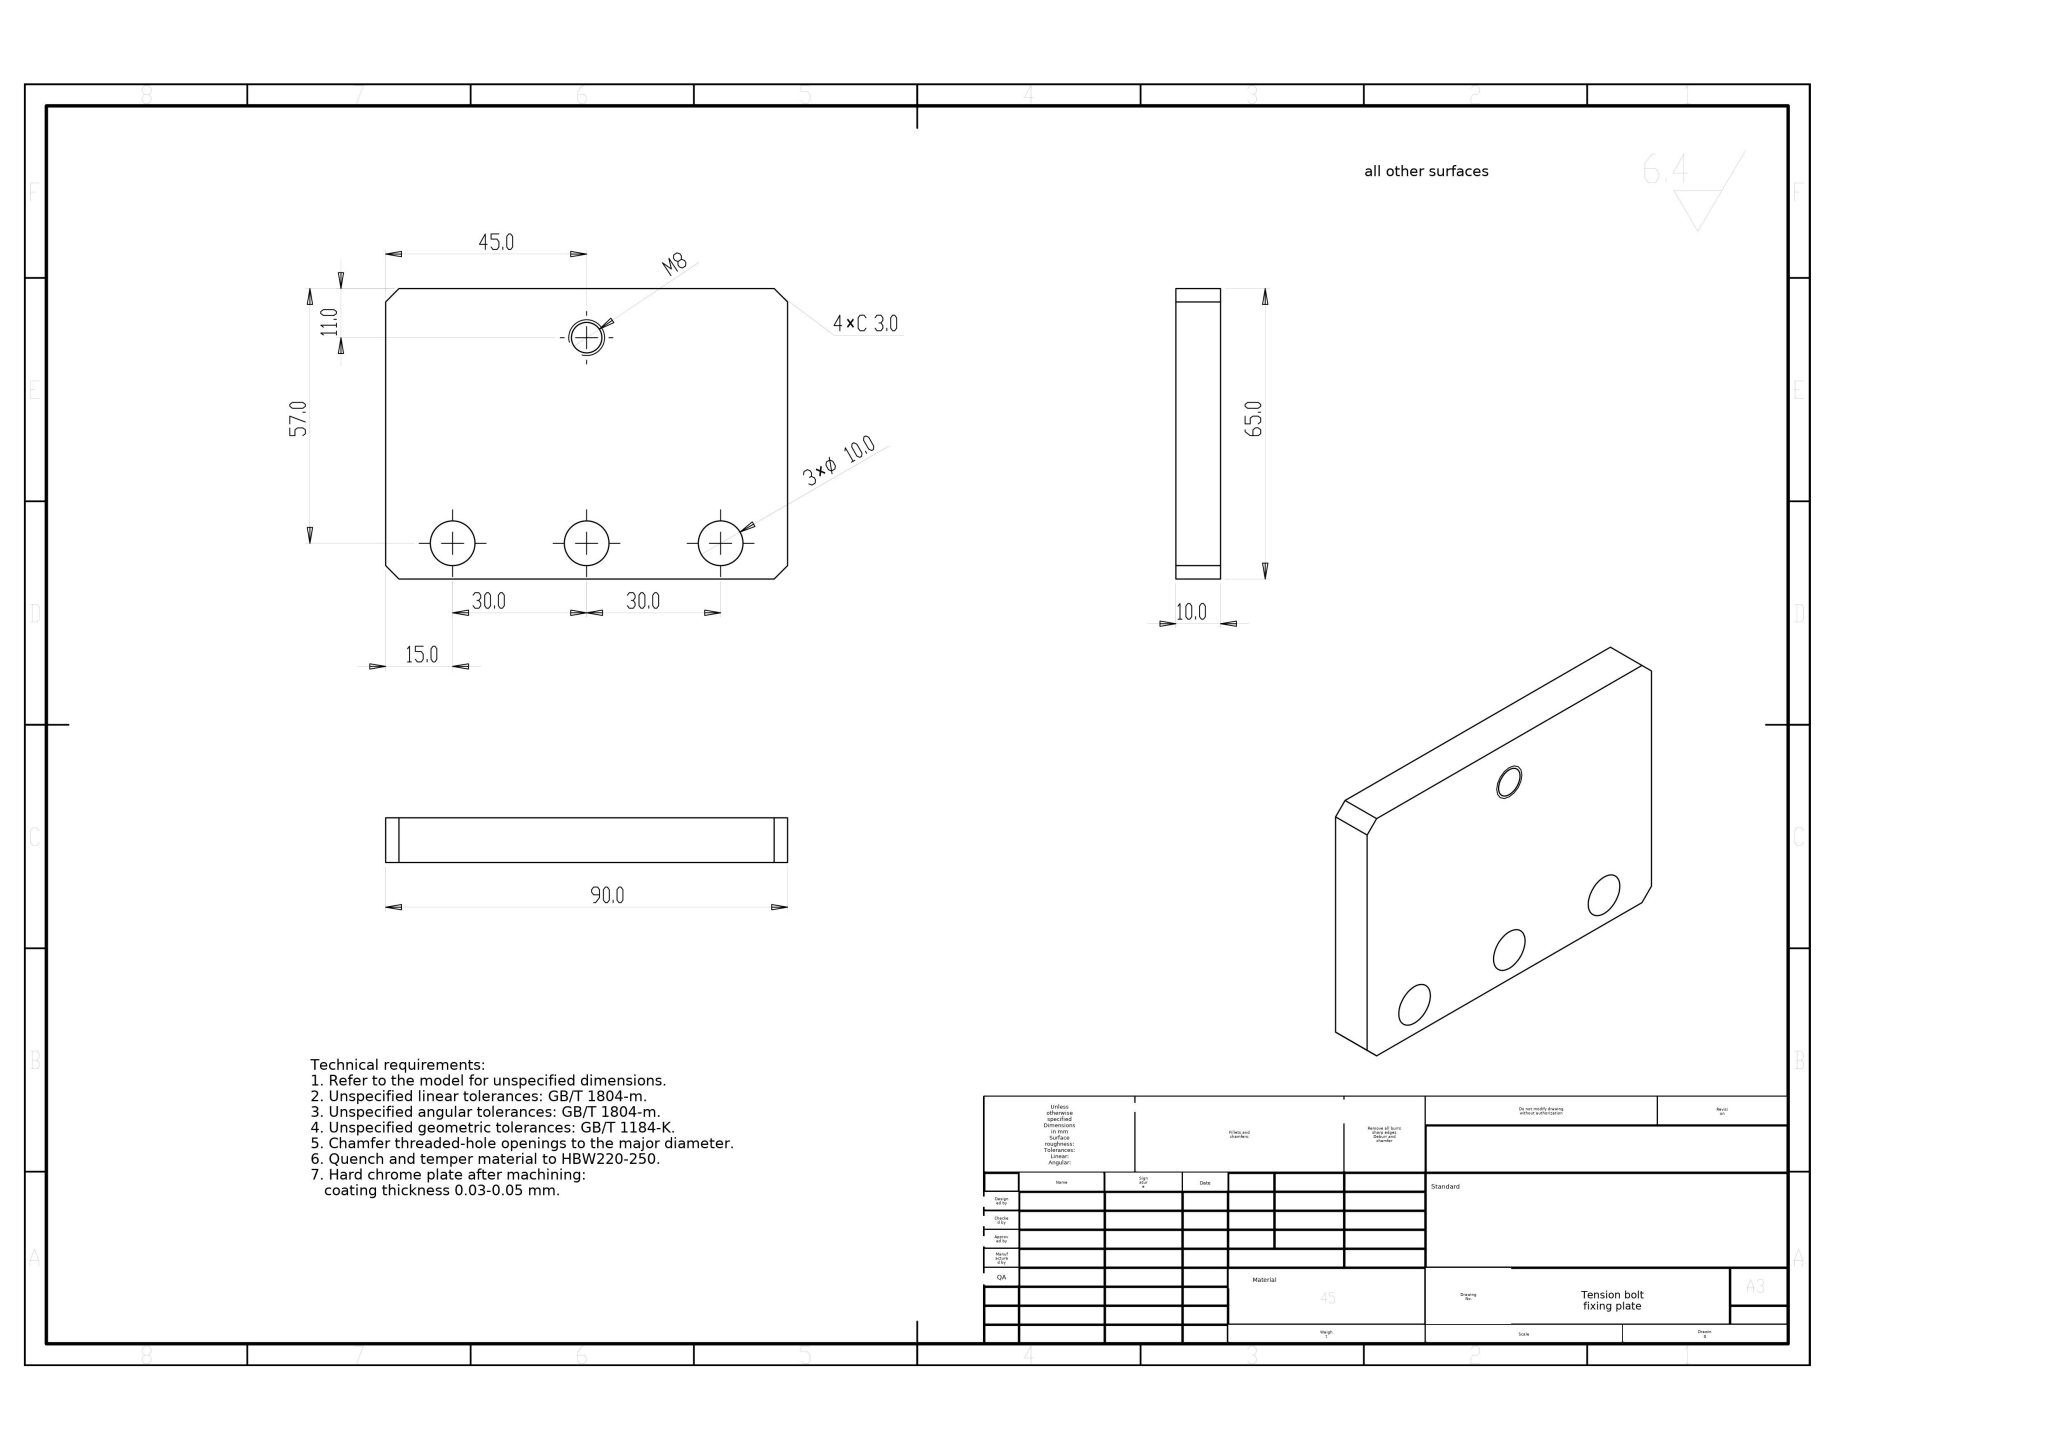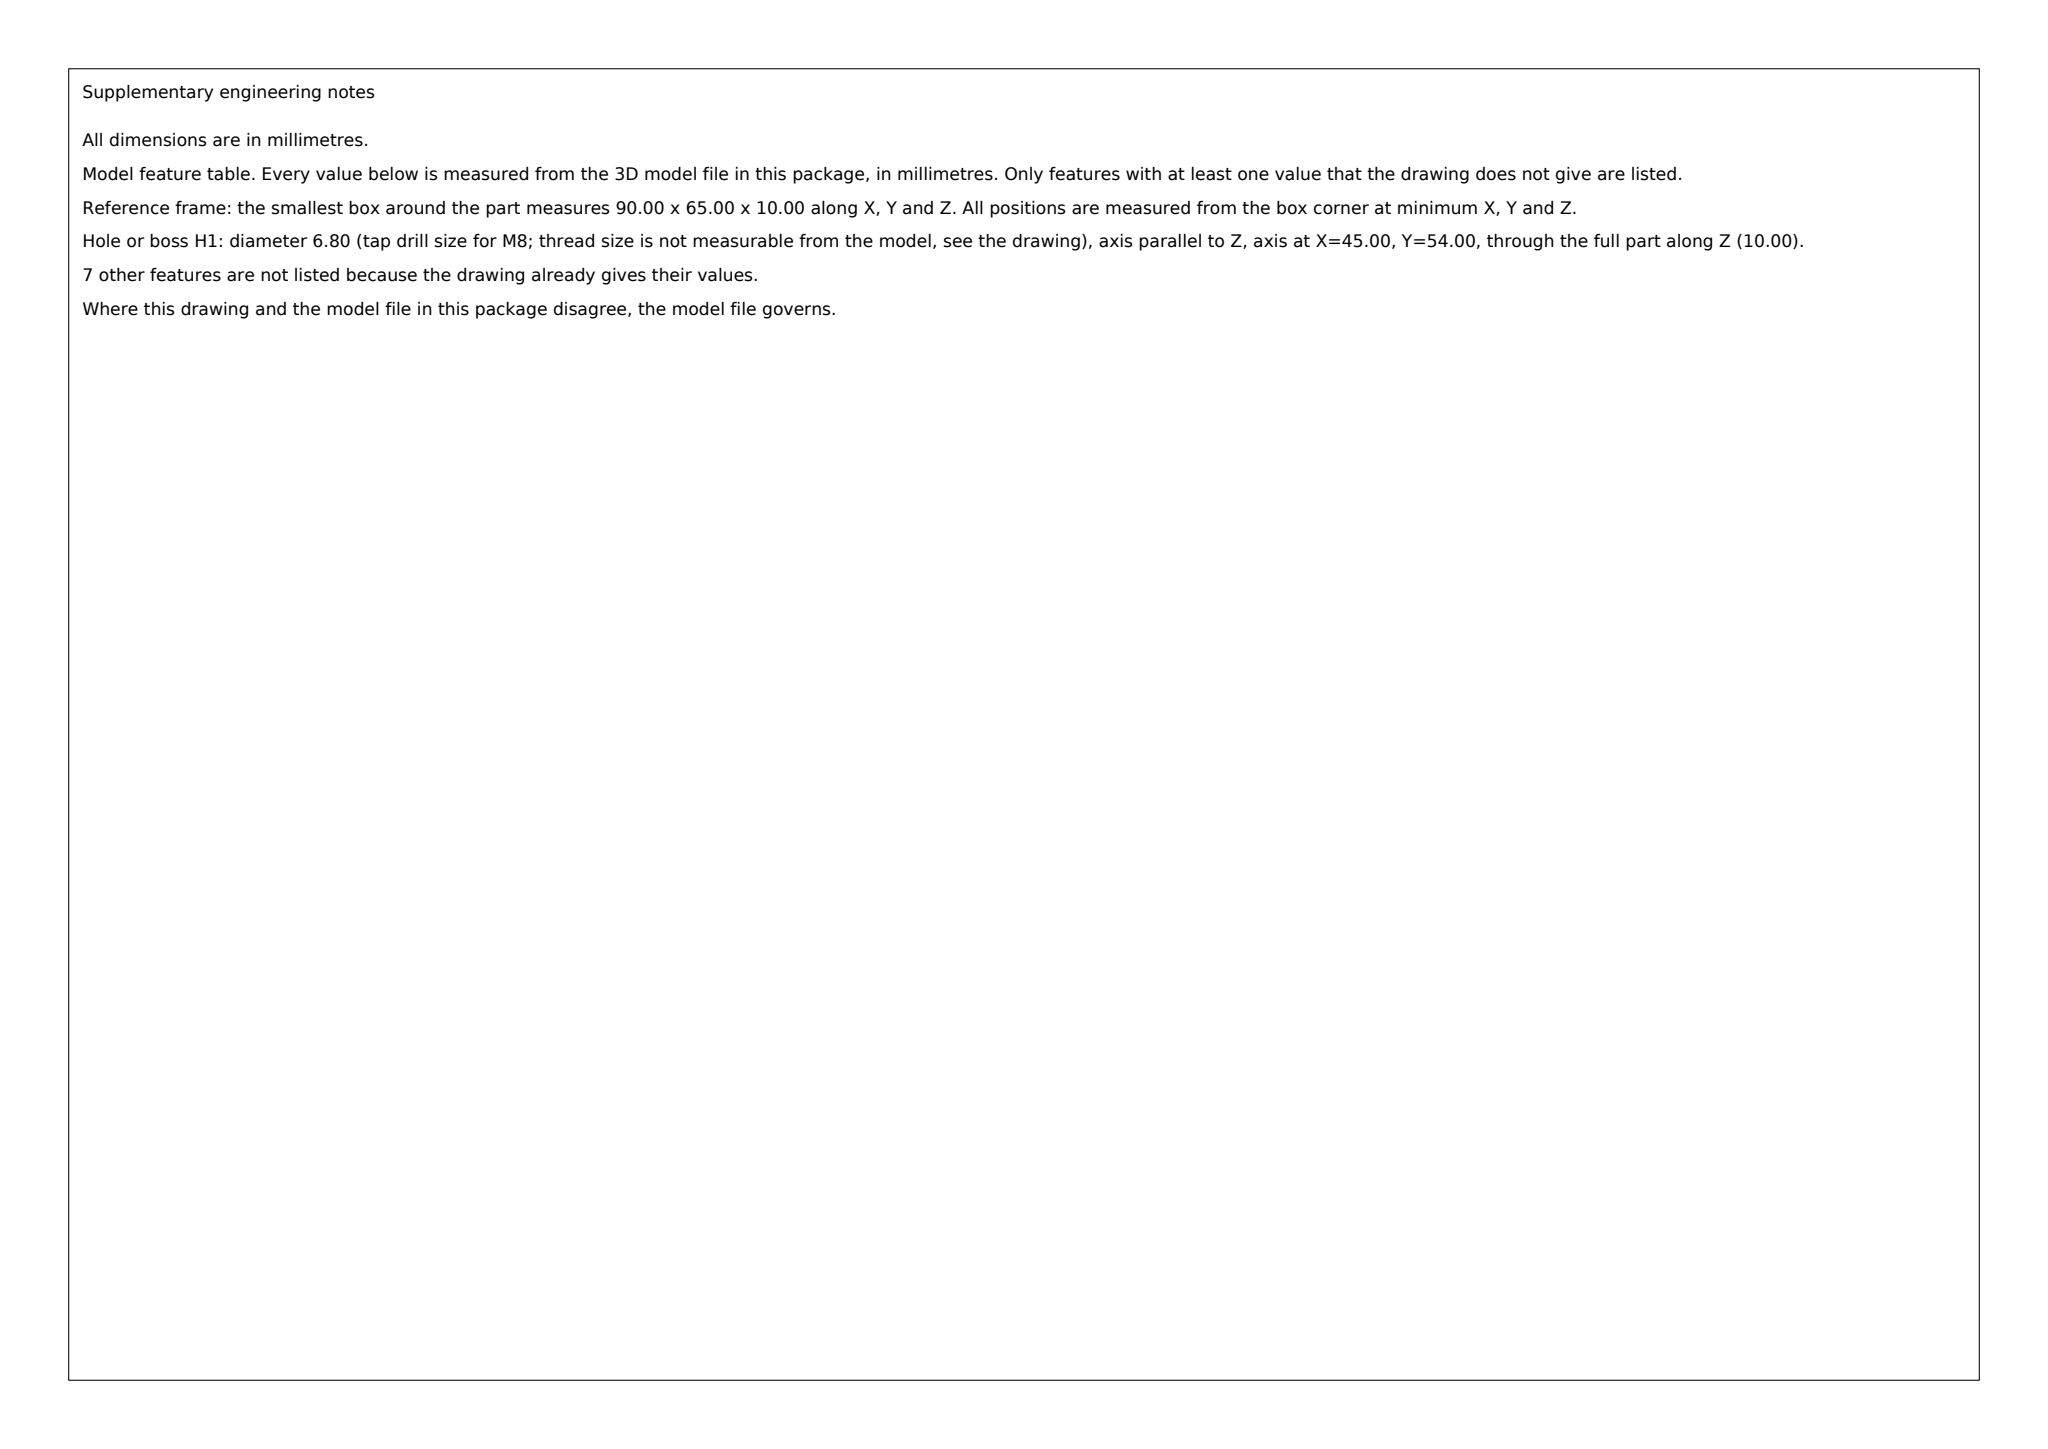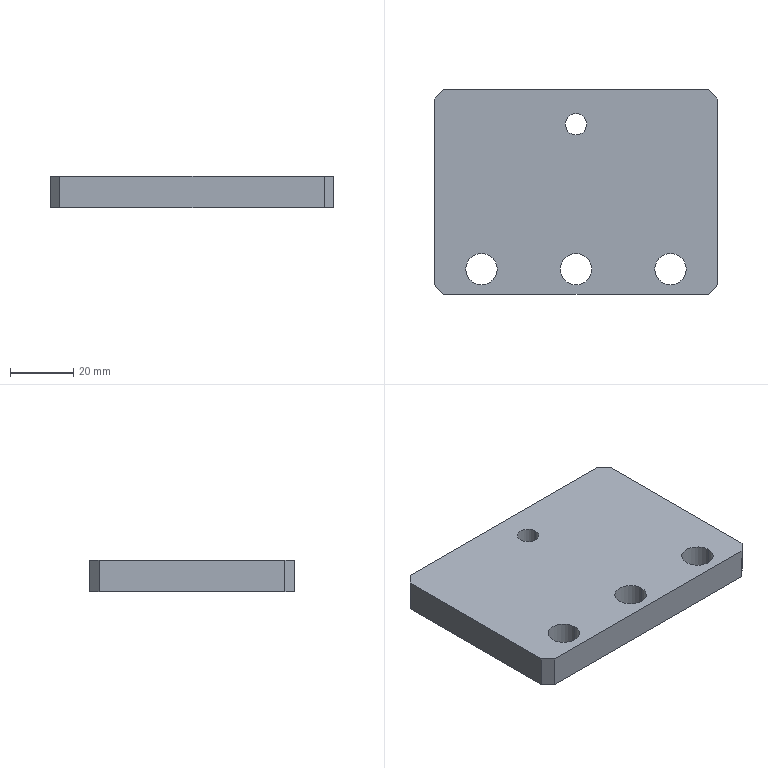Part | SolidWorks | mm | material 45 | 1 solid | 18 faces | box 90 x 65 x 10 mm | volume 55601 mm3 | plane 10 | cylinder 8 | commonest cylinder face diameters 10 x6 6.8 x2
build123d program:
from build123d import *

# Parameters (mm, degrees)
SKETCH1_W           = 90
SKETCH1_H           = 65
SKETCH1_R           = 5
BOSS_EXTRUDE1_DEPTH = 10
M8_TAPPED_HOLE1_D   = 6.8
CHAMFER1_SIZE       = 3


with BuildPart() as part:
    # Sketch1 → Boss-Extrude1 (new body)
    with BuildSketch(Plane.XY):
        with Locations((0, 24.5)):
            Rectangle(SKETCH1_W, SKETCH1_H)
        Circle(SKETCH1_R, mode=Mode.SUBTRACT)
        with Locations((30, 0)):
            Circle(SKETCH1_R, mode=Mode.SUBTRACT)
        with Locations(Location((-30, 0, 0), (0, 0, 180))):
            Circle(SKETCH1_R, mode=Mode.SUBTRACT)
    extrude(amount=BOSS_EXTRUDE1_DEPTH)

    # M8 Tapped Hole1 (through all)
    with Locations(Plane.XY.offset(10)):
        with Locations((0, 46)):
            Hole(M8_TAPPED_HOLE1_D / 2)

    # Chamfer1
    chamfer1_edges = [part.edges().sort_by_distance(p)[0] for p in [
        (45, -8, 5),
        (-45, -8, 5),
        (-45, 57, 5),
        (45, 57, 5),
    ]]
    chamfer(chamfer1_edges, length=CHAMFER1_SIZE)


solid = part.part
STEP:
#1=CARTESIAN_POINT('',(-3.4,46.,0.));
#2=VERTEX_POINT('',#1);
#3=CARTESIAN_POINT('',(3.4,46.,0.));
#4=VERTEX_POINT('',#3);
#5=CARTESIAN_POINT('',(0.,46.,0.));
#6=DIRECTION('',(0.,0.,1.));
#7=DIRECTION('',(1.,0.,0.));
#8=AXIS2_PLACEMENT_3D('',#5,#6,#7);
#9=CIRCLE('',#8,3.4);
#10=EDGE_CURVE('',#2,#4,#9,.T.);
#11=ORIENTED_EDGE('',*,*,#10,.F.);
#12=CARTESIAN_POINT('',(-3.4,46.,10.));
#13=VERTEX_POINT('',#12);
#14=CARTESIAN_POINT('',(-3.4,46.,10.));
#15=DIRECTION('',(0.,0.,1.));
#16=VECTOR('',#15,1000.);
#17=LINE('',#14,#16);
#18=EDGE_CURVE('',#2,#13,#17,.T.);
#19=ORIENTED_EDGE('',*,*,#18,.T.);
#20=CARTESIAN_POINT('',(3.4,46.,10.));
#21=VERTEX_POINT('',#20);
#22=CARTESIAN_POINT('',(0.,46.,10.));
#23=DIRECTION('',(0.,0.,1.));
#24=DIRECTION('',(1.,0.,0.));
#25=AXIS2_PLACEMENT_3D('',#22,#23,#24);
#26=CIRCLE('',#25,3.4);
#27=EDGE_CURVE('',#13,#21,#26,.T.);
#28=ORIENTED_EDGE('',*,*,#27,.T.);
#29=CARTESIAN_POINT('',(3.4,46.,10.));
#30=DIRECTION('',(0.,0.,1.));
#31=VECTOR('',#30,1000.);
#32=LINE('',#29,#31);
#33=EDGE_CURVE('',#4,#21,#32,.T.);
#34=ORIENTED_EDGE('',*,*,#33,.F.);
#35=EDGE_LOOP('',(#11,#19,#28,#34));
#36=FACE_OUTER_BOUND('',#35,.T.);
#37=CARTESIAN_POINT('',(0.,46.,10.));
#38=DIRECTION('',(0.,0.,1.));
#39=DIRECTION('',(1.,0.,0.));
#40=AXIS2_PLACEMENT_3D('',#37,#38,#39);
#41=CYLINDRICAL_SURFACE('',#40,3.4);
#42=ADVANCED_FACE('',(#36),#41,.F.);
#43=CARTESIAN_POINT('',(-35.,-0.,10.));
#44=VERTEX_POINT('',#43);
#45=CARTESIAN_POINT('',(-25.,-0.,10.));
#46=VERTEX_POINT('',#45);
#47=CARTESIAN_POINT('',(-30.,-0.,10.));
#48=DIRECTION('',(0.,0.,1.));
#49=DIRECTION('',(-1.,0.,0.));
#50=AXIS2_PLACEMENT_3D('',#47,#48,#49);
#51=CIRCLE('',#50,5.);
#52=EDGE_CURVE('',#44,#46,#51,.T.);
#53=ORIENTED_EDGE('',*,*,#52,.T.);
#54=CARTESIAN_POINT('',(-25.,-0.,0.));
#55=VERTEX_POINT('',#54);
#56=CARTESIAN_POINT('',(-25.,-0.,10.));
#57=DIRECTION('',(0.,0.,-1.));
#58=VECTOR('',#57,1000.);
#59=LINE('',#56,#58);
#60=EDGE_CURVE('',#46,#55,#59,.T.);
#61=ORIENTED_EDGE('',*,*,#60,.T.);
#62=CARTESIAN_POINT('',(-35.,-0.,0.));
#63=VERTEX_POINT('',#62);
#64=CARTESIAN_POINT('',(-30.,-0.,0.));
#65=DIRECTION('',(0.,0.,1.));
#66=DIRECTION('',(-1.,0.,0.));
#67=AXIS2_PLACEMENT_3D('',#64,#65,#66);
#68=CIRCLE('',#67,5.);
#69=EDGE_CURVE('',#63,#55,#68,.T.);
#70=ORIENTED_EDGE('',*,*,#69,.F.);
#71=CARTESIAN_POINT('',(-35.,-0.,10.));
#72=DIRECTION('',(0.,0.,-1.));
#73=VECTOR('',#72,1000.);
#74=LINE('',#71,#73);
#75=EDGE_CURVE('',#44,#63,#74,.T.);
#76=ORIENTED_EDGE('',*,*,#75,.F.);
#77=EDGE_LOOP('',(#53,#61,#70,#76));
#78=FACE_OUTER_BOUND('',#77,.T.);
#79=CARTESIAN_POINT('',(-30.,-0.,10.));
#80=DIRECTION('',(0.,0.,-1.));
#81=DIRECTION('',(-1.,0.,0.));
#82=AXIS2_PLACEMENT_3D('',#79,#80,#81);
#83=CYLINDRICAL_SURFACE('',#82,5.);
#84=ADVANCED_FACE('',(#78),#83,.F.);
#85=CARTESIAN_POINT('',(25.,0.,10.));
#86=VERTEX_POINT('',#85);
#87=CARTESIAN_POINT('',(35.,0.,10.));
#88=VERTEX_POINT('',#87);
#89=CARTESIAN_POINT('',(30.,0.,10.));
#90=DIRECTION('',(0.,0.,1.));
#91=DIRECTION('',(1.,0.,0.));
#92=AXIS2_PLACEMENT_3D('',#89,#90,#91);
#93=CIRCLE('',#92,5.);
#94=EDGE_CURVE('',#86,#88,#93,.T.);
#95=ORIENTED_EDGE('',*,*,#94,.T.);
#96=CARTESIAN_POINT('',(35.,0.,0.));
#97=VERTEX_POINT('',#96);
#98=CARTESIAN_POINT('',(35.,0.,10.));
#99=DIRECTION('',(0.,0.,-1.));
#100=VECTOR('',#99,1000.);
#101=LINE('',#98,#100);
#102=EDGE_CURVE('',#88,#97,#101,.T.);
#103=ORIENTED_EDGE('',*,*,#102,.T.);
#104=CARTESIAN_POINT('',(25.,0.,0.));
#105=VERTEX_POINT('',#104);
#106=CARTESIAN_POINT('',(30.,0.,0.));
#107=DIRECTION('',(0.,0.,1.));
#108=DIRECTION('',(1.,0.,0.));
#109=AXIS2_PLACEMENT_3D('',#106,#107,#108);
#110=CIRCLE('',#109,5.);
#111=EDGE_CURVE('',#105,#97,#110,.T.);
#112=ORIENTED_EDGE('',*,*,#111,.F.);
#113=CARTESIAN_POINT('',(25.,0.,10.));
#114=DIRECTION('',(0.,0.,-1.));
#115=VECTOR('',#114,1000.);
#116=LINE('',#113,#115);
#117=EDGE_CURVE('',#86,#105,#116,.T.);
#118=ORIENTED_EDGE('',*,*,#117,.F.);
#119=EDGE_LOOP('',(#95,#103,#112,#118));
#120=FACE_OUTER_BOUND('',#119,.T.);
#121=CARTESIAN_POINT('',(30.,0.,10.));
#122=DIRECTION('',(0.,0.,-1.));
#123=DIRECTION('',(-1.,0.,0.));
#124=AXIS2_PLACEMENT_3D('',#121,#122,#123);
#125=CYLINDRICAL_SURFACE('',#124,5.);
#126=ADVANCED_FACE('',(#120),#125,.F.);
#127=CARTESIAN_POINT('',(-5.,0.,10.));
#128=VERTEX_POINT('',#127);
#129=CARTESIAN_POINT('',(5.,0.,10.));
#130=VERTEX_POINT('',#129);
#131=CARTESIAN_POINT('',(0.,0.,10.));
#132=DIRECTION('',(0.,0.,1.));
#133=DIRECTION('',(1.,0.,0.));
#134=AXIS2_PLACEMENT_3D('',#131,#132,#133);
#135=CIRCLE('',#134,5.);
#136=EDGE_CURVE('',#128,#130,#135,.T.);
#137=ORIENTED_EDGE('',*,*,#136,.T.);
#138=CARTESIAN_POINT('',(5.,0.,0.));
#139=VERTEX_POINT('',#138);
#140=CARTESIAN_POINT('',(5.,0.,10.));
#141=DIRECTION('',(0.,0.,-1.));
#142=VECTOR('',#141,1000.);
#143=LINE('',#140,#142);
#144=EDGE_CURVE('',#130,#139,#143,.T.);
#145=ORIENTED_EDGE('',*,*,#144,.T.);
#146=CARTESIAN_POINT('',(-5.,0.,0.));
#147=VERTEX_POINT('',#146);
#148=CARTESIAN_POINT('',(0.,0.,0.));
#149=DIRECTION('',(0.,0.,1.));
#150=DIRECTION('',(1.,0.,0.));
#151=AXIS2_PLACEMENT_3D('',#148,#149,#150);
#152=CIRCLE('',#151,5.);
#153=EDGE_CURVE('',#147,#139,#152,.T.);
#154=ORIENTED_EDGE('',*,*,#153,.F.);
#155=CARTESIAN_POINT('',(-5.,0.,10.));
#156=DIRECTION('',(0.,0.,-1.));
#157=VECTOR('',#156,1000.);
#158=LINE('',#155,#157);
#159=EDGE_CURVE('',#128,#147,#158,.T.);
#160=ORIENTED_EDGE('',*,*,#159,.F.);
#161=EDGE_LOOP('',(#137,#145,#154,#160));
#162=FACE_OUTER_BOUND('',#161,.T.);
#163=CARTESIAN_POINT('',(0.,0.,10.));
#164=DIRECTION('',(0.,0.,-1.));
#165=DIRECTION('',(-1.,0.,0.));
#166=AXIS2_PLACEMENT_3D('',#163,#164,#165);
#167=CYLINDRICAL_SURFACE('',#166,5.);
#168=ADVANCED_FACE('',(#162),#167,.F.);
#169=CARTESIAN_POINT('',(0.,46.,10.));
#170=DIRECTION('',(0.,0.,1.));
#171=DIRECTION('',(1.,0.,0.));
#172=AXIS2_PLACEMENT_3D('',#169,#170,#171);
#173=CIRCLE('',#172,3.4);
#174=EDGE_CURVE('',#21,#13,#173,.T.);
#175=ORIENTED_EDGE('',*,*,#174,.F.);
#176=ORIENTED_EDGE('',*,*,#27,.F.);
#177=EDGE_LOOP('',(#175,#176));
#178=FACE_BOUND('',#177,.T.);
#179=ORIENTED_EDGE('',*,*,#94,.F.);
#180=CARTESIAN_POINT('',(30.,0.,10.));
#181=DIRECTION('',(0.,0.,1.));
#182=DIRECTION('',(1.,0.,0.));
#183=AXIS2_PLACEMENT_3D('',#180,#181,#182);
#184=CIRCLE('',#183,5.);
#185=EDGE_CURVE('',#88,#86,#184,.T.);
#186=ORIENTED_EDGE('',*,*,#185,.F.);
#187=EDGE_LOOP('',(#179,#186));
#188=FACE_BOUND('',#187,.T.);
#189=CARTESIAN_POINT('',(42.,57.,10.));
#190=VERTEX_POINT('',#189);
#191=CARTESIAN_POINT('',(-42.,57.,10.));
#192=VERTEX_POINT('',#191);
#193=CARTESIAN_POINT('',(-45.,57.,10.));
#194=DIRECTION('',(-1.,0.,0.));
#195=VECTOR('',#194,1000.);
#196=LINE('',#193,#195);
#197=EDGE_CURVE('',#190,#192,#196,.T.);
#198=ORIENTED_EDGE('',*,*,#197,.T.);
#199=CARTESIAN_POINT('',(-45.,54.,10.));
#200=VERTEX_POINT('',#199);
#201=CARTESIAN_POINT('',(-49.5,49.5,10.));
#202=DIRECTION('',(-0.7071,-0.7071,0.));
#203=VECTOR('',#202,1000.);
#204=LINE('',#201,#203);
#205=EDGE_CURVE('',#192,#200,#204,.T.);
#206=ORIENTED_EDGE('',*,*,#205,.T.);
#207=CARTESIAN_POINT('',(-45.,-5.,10.));
#208=VERTEX_POINT('',#207);
#209=CARTESIAN_POINT('',(-45.,57.,10.));
#210=DIRECTION('',(0.,-1.,0.));
#211=VECTOR('',#210,1000.);
#212=LINE('',#209,#211);
#213=EDGE_CURVE('',#200,#208,#212,.T.);
#214=ORIENTED_EDGE('',*,*,#213,.T.);
#215=CARTESIAN_POINT('',(-42.,-8.,10.));
#216=VERTEX_POINT('',#215);
#217=CARTESIAN_POINT('',(-25.,-25.,10.));
#218=DIRECTION('',(0.7071,-0.7071,0.));
#219=VECTOR('',#218,1000.);
#220=LINE('',#217,#219);
#221=EDGE_CURVE('',#208,#216,#220,.T.);
#222=ORIENTED_EDGE('',*,*,#221,.T.);
#223=CARTESIAN_POINT('',(42.,-8.,10.));
#224=VERTEX_POINT('',#223);
#225=CARTESIAN_POINT('',(-45.,-8.,10.));
#226=DIRECTION('',(1.,0.,0.));
#227=VECTOR('',#226,1000.);
#228=LINE('',#225,#227);
#229=EDGE_CURVE('',#216,#224,#228,.T.);
#230=ORIENTED_EDGE('',*,*,#229,.T.);
#231=CARTESIAN_POINT('',(45.,-5.,10.));
#232=VERTEX_POINT('',#231);
#233=CARTESIAN_POINT('',(25.,-25.,10.));
#234=DIRECTION('',(0.7071,0.7071,0.));
#235=VECTOR('',#234,1000.);
#236=LINE('',#233,#235);
#237=EDGE_CURVE('',#224,#232,#236,.T.);
#238=ORIENTED_EDGE('',*,*,#237,.T.);
#239=CARTESIAN_POINT('',(45.,54.,10.));
#240=VERTEX_POINT('',#239);
#241=CARTESIAN_POINT('',(45.,57.,10.));
#242=DIRECTION('',(0.,1.,0.));
#243=VECTOR('',#242,1000.);
#244=LINE('',#241,#243);
#245=EDGE_CURVE('',#232,#240,#244,.T.);
#246=ORIENTED_EDGE('',*,*,#245,.T.);
#247=CARTESIAN_POINT('',(49.5,49.5,10.));
#248=DIRECTION('',(-0.7071,0.7071,0.));
#249=VECTOR('',#248,1000.);
#250=LINE('',#247,#249);
#251=EDGE_CURVE('',#240,#190,#250,.T.);
#252=ORIENTED_EDGE('',*,*,#251,.T.);
#253=EDGE_LOOP('',(#198,#206,#214,#222,#230,#238,#246,#252));
#254=FACE_OUTER_BOUND('',#253,.T.);
#255=ORIENTED_EDGE('',*,*,#136,.F.);
#256=CARTESIAN_POINT('',(0.,0.,10.));
#257=DIRECTION('',(0.,0.,1.));
#258=DIRECTION('',(1.,0.,0.));
#259=AXIS2_PLACEMENT_3D('',#256,#257,#258);
#260=CIRCLE('',#259,5.);
#261=EDGE_CURVE('',#130,#128,#260,.T.);
#262=ORIENTED_EDGE('',*,*,#261,.F.);
#263=EDGE_LOOP('',(#255,#262));
#264=FACE_BOUND('',#263,.T.);
#265=ORIENTED_EDGE('',*,*,#52,.F.);
#266=CARTESIAN_POINT('',(-30.,-0.,10.));
#267=DIRECTION('',(0.,0.,1.));
#268=DIRECTION('',(-1.,0.,0.));
#269=AXIS2_PLACEMENT_3D('',#266,#267,#268);
#270=CIRCLE('',#269,5.);
#271=EDGE_CURVE('',#46,#44,#270,.T.);
#272=ORIENTED_EDGE('',*,*,#271,.F.);
#273=EDGE_LOOP('',(#265,#272));
#274=FACE_BOUND('',#273,.T.);
#275=CARTESIAN_POINT('',(0.,0.,10.));
#276=DIRECTION('',(0.,0.,1.));
#277=DIRECTION('',(1.,0.,0.));
#278=AXIS2_PLACEMENT_3D('',#275,#276,#277);
#279=PLANE('',#278);
#280=ADVANCED_FACE('',(#178,#188,#254,#264,#274),#279,.T.);
#281=CARTESIAN_POINT('',(0.,46.,0.));
#282=DIRECTION('',(0.,0.,1.));
#283=DIRECTION('',(1.,0.,0.));
#284=AXIS2_PLACEMENT_3D('',#281,#282,#283);
#285=CIRCLE('',#284,3.4);
#286=EDGE_CURVE('',#4,#2,#285,.T.);
#287=ORIENTED_EDGE('',*,*,#286,.T.);
#288=ORIENTED_EDGE('',*,*,#10,.T.);
#289=EDGE_LOOP('',(#287,#288));
#290=FACE_BOUND('',#289,.T.);
#291=CARTESIAN_POINT('',(-45.,54.,0.));
#292=VERTEX_POINT('',#291);
#293=CARTESIAN_POINT('',(-45.,-5.,0.));
#294=VERTEX_POINT('',#293);
#295=CARTESIAN_POINT('',(-45.,57.,0.));
#296=DIRECTION('',(0.,-1.,0.));
#297=VECTOR('',#296,1000.);
#298=LINE('',#295,#297);
#299=EDGE_CURVE('',#292,#294,#298,.T.);
#300=ORIENTED_EDGE('',*,*,#299,.F.);
#301=CARTESIAN_POINT('',(-42.,57.,0.));
#302=VERTEX_POINT('',#301);
#303=CARTESIAN_POINT('',(-45.,54.,0.));
#304=DIRECTION('',(0.7071,0.7071,0.));
#305=VECTOR('',#304,1000.);
#306=LINE('',#303,#305);
#307=EDGE_CURVE('',#292,#302,#306,.T.);
#308=ORIENTED_EDGE('',*,*,#307,.T.);
#309=CARTESIAN_POINT('',(42.,57.,0.));
#310=VERTEX_POINT('',#309);
#311=CARTESIAN_POINT('',(-45.,57.,0.));
#312=DIRECTION('',(-1.,0.,0.));
#313=VECTOR('',#312,1000.);
#314=LINE('',#311,#313);
#315=EDGE_CURVE('',#310,#302,#314,.T.);
#316=ORIENTED_EDGE('',*,*,#315,.F.);
#317=CARTESIAN_POINT('',(45.,54.,0.));
#318=VERTEX_POINT('',#317);
#319=CARTESIAN_POINT('',(42.,57.,0.));
#320=DIRECTION('',(0.7071,-0.7071,0.));
#321=VECTOR('',#320,1000.);
#322=LINE('',#319,#321);
#323=EDGE_CURVE('',#310,#318,#322,.T.);
#324=ORIENTED_EDGE('',*,*,#323,.T.);
#325=CARTESIAN_POINT('',(45.,-5.,0.));
#326=VERTEX_POINT('',#325);
#327=CARTESIAN_POINT('',(45.,57.,0.));
#328=DIRECTION('',(0.,1.,0.));
#329=VECTOR('',#328,1000.);
#330=LINE('',#327,#329);
#331=EDGE_CURVE('',#326,#318,#330,.T.);
#332=ORIENTED_EDGE('',*,*,#331,.F.);
#333=CARTESIAN_POINT('',(42.,-8.,0.));
#334=VERTEX_POINT('',#333);
#335=CARTESIAN_POINT('',(45.,-5.,0.));
#336=DIRECTION('',(-0.7071,-0.7071,0.));
#337=VECTOR('',#336,1000.);
#338=LINE('',#335,#337);
#339=EDGE_CURVE('',#326,#334,#338,.T.);
#340=ORIENTED_EDGE('',*,*,#339,.T.);
#341=CARTESIAN_POINT('',(-42.,-8.,0.));
#342=VERTEX_POINT('',#341);
#343=CARTESIAN_POINT('',(-45.,-8.,0.));
#344=DIRECTION('',(1.,0.,0.));
#345=VECTOR('',#344,1000.);
#346=LINE('',#343,#345);
#347=EDGE_CURVE('',#342,#334,#346,.T.);
#348=ORIENTED_EDGE('',*,*,#347,.F.);
#349=CARTESIAN_POINT('',(-42.,-8.,0.));
#350=DIRECTION('',(-0.7071,0.7071,0.));
#351=VECTOR('',#350,1000.);
#352=LINE('',#349,#351);
#353=EDGE_CURVE('',#342,#294,#352,.T.);
#354=ORIENTED_EDGE('',*,*,#353,.T.);
#355=EDGE_LOOP('',(#300,#308,#316,#324,#332,#340,#348,#354));
#356=FACE_OUTER_BOUND('',#355,.T.);
#357=ORIENTED_EDGE('',*,*,#153,.T.);
#358=CARTESIAN_POINT('',(0.,0.,0.));
#359=DIRECTION('',(0.,0.,1.));
#360=DIRECTION('',(1.,0.,0.));
#361=AXIS2_PLACEMENT_3D('',#358,#359,#360);
#362=CIRCLE('',#361,5.);
#363=EDGE_CURVE('',#139,#147,#362,.T.);
#364=ORIENTED_EDGE('',*,*,#363,.T.);
#365=EDGE_LOOP('',(#357,#364));
#366=FACE_BOUND('',#365,.T.);
#367=ORIENTED_EDGE('',*,*,#111,.T.);
#368=CARTESIAN_POINT('',(30.,0.,0.));
#369=DIRECTION('',(0.,0.,1.));
#370=DIRECTION('',(1.,0.,0.));
#371=AXIS2_PLACEMENT_3D('',#368,#369,#370);
#372=CIRCLE('',#371,5.);
#373=EDGE_CURVE('',#97,#105,#372,.T.);
#374=ORIENTED_EDGE('',*,*,#373,.T.);
#375=EDGE_LOOP('',(#367,#374));
#376=FACE_BOUND('',#375,.T.);
#377=ORIENTED_EDGE('',*,*,#69,.T.);
#378=CARTESIAN_POINT('',(-30.,-0.,0.));
#379=DIRECTION('',(0.,0.,1.));
#380=DIRECTION('',(-1.,0.,0.));
#381=AXIS2_PLACEMENT_3D('',#378,#379,#380);
#382=CIRCLE('',#381,5.);
#383=EDGE_CURVE('',#55,#63,#382,.T.);
#384=ORIENTED_EDGE('',*,*,#383,.T.);
#385=EDGE_LOOP('',(#377,#384));
#386=FACE_BOUND('',#385,.T.);
#387=CARTESIAN_POINT('',(0.,0.,0.));
#388=DIRECTION('',(0.,0.,1.));
#389=DIRECTION('',(1.,0.,0.));
#390=AXIS2_PLACEMENT_3D('',#387,#388,#389);
#391=PLANE('',#390);
#392=ADVANCED_FACE('',(#290,#356,#366,#376,#386),#391,.F.);
#393=ORIENTED_EDGE('',*,*,#331,.T.);
#394=CARTESIAN_POINT('',(45.,54.,10.));
#395=DIRECTION('',(0.,0.,1.));
#396=VECTOR('',#395,1000.);
#397=LINE('',#394,#396);
#398=EDGE_CURVE('',#318,#240,#397,.T.);
#399=ORIENTED_EDGE('',*,*,#398,.T.);
#400=ORIENTED_EDGE('',*,*,#245,.F.);
#401=CARTESIAN_POINT('',(45.,-5.,10.));
#402=DIRECTION('',(0.,0.,-1.));
#403=VECTOR('',#402,1000.);
#404=LINE('',#401,#403);
#405=EDGE_CURVE('',#232,#326,#404,.T.);
#406=ORIENTED_EDGE('',*,*,#405,.T.);
#407=EDGE_LOOP('',(#393,#399,#400,#406));
#408=FACE_OUTER_BOUND('',#407,.T.);
#409=CARTESIAN_POINT('',(45.,57.,10.));
#410=DIRECTION('',(-1.,0.,0.));
#411=DIRECTION('',(0.,0.,1.));
#412=AXIS2_PLACEMENT_3D('',#409,#410,#411);
#413=PLANE('',#412);
#414=ADVANCED_FACE('',(#408),#413,.F.);
#415=ORIENTED_EDGE('',*,*,#315,.T.);
#416=CARTESIAN_POINT('',(-42.,57.,10.));
#417=DIRECTION('',(0.,0.,1.));
#418=VECTOR('',#417,1000.);
#419=LINE('',#416,#418);
#420=EDGE_CURVE('',#302,#192,#419,.T.);
#421=ORIENTED_EDGE('',*,*,#420,.T.);
#422=ORIENTED_EDGE('',*,*,#197,.F.);
#423=CARTESIAN_POINT('',(42.,57.,10.));
#424=DIRECTION('',(0.,0.,-1.));
#425=VECTOR('',#424,1000.);
#426=LINE('',#423,#425);
#427=EDGE_CURVE('',#190,#310,#426,.T.);
#428=ORIENTED_EDGE('',*,*,#427,.T.);
#429=EDGE_LOOP('',(#415,#421,#422,#428));
#430=FACE_OUTER_BOUND('',#429,.T.);
#431=CARTESIAN_POINT('',(-45.,57.,10.));
#432=DIRECTION('',(0.,-1.,0.));
#433=DIRECTION('',(0.,0.,-1.));
#434=AXIS2_PLACEMENT_3D('',#431,#432,#433);
#435=PLANE('',#434);
#436=ADVANCED_FACE('',(#430),#435,.F.);
#437=ORIENTED_EDGE('',*,*,#213,.F.);
#438=CARTESIAN_POINT('',(-45.,54.,10.));
#439=DIRECTION('',(0.,0.,-1.));
#440=VECTOR('',#439,1000.);
#441=LINE('',#438,#440);
#442=EDGE_CURVE('',#200,#292,#441,.T.);
#443=ORIENTED_EDGE('',*,*,#442,.T.);
#444=ORIENTED_EDGE('',*,*,#299,.T.);
#445=CARTESIAN_POINT('',(-45.,-5.,10.));
#446=DIRECTION('',(0.,0.,1.));
#447=VECTOR('',#446,1000.);
#448=LINE('',#445,#447);
#449=EDGE_CURVE('',#294,#208,#448,.T.);
#450=ORIENTED_EDGE('',*,*,#449,.T.);
#451=EDGE_LOOP('',(#437,#443,#444,#450));
#452=FACE_OUTER_BOUND('',#451,.T.);
#453=CARTESIAN_POINT('',(-45.,57.,10.));
#454=DIRECTION('',(1.,0.,0.));
#455=DIRECTION('',(-0.,1.,0.));
#456=AXIS2_PLACEMENT_3D('',#453,#454,#455);
#457=PLANE('',#456);
#458=ADVANCED_FACE('',(#452),#457,.F.);
#459=ORIENTED_EDGE('',*,*,#347,.T.);
#460=CARTESIAN_POINT('',(42.,-8.,10.));
#461=DIRECTION('',(0.,0.,1.));
#462=VECTOR('',#461,1000.);
#463=LINE('',#460,#462);
#464=EDGE_CURVE('',#334,#224,#463,.T.);
#465=ORIENTED_EDGE('',*,*,#464,.T.);
#466=ORIENTED_EDGE('',*,*,#229,.F.);
#467=CARTESIAN_POINT('',(-42.,-8.,10.));
#468=DIRECTION('',(0.,0.,-1.));
#469=VECTOR('',#468,1000.);
#470=LINE('',#467,#469);
#471=EDGE_CURVE('',#216,#342,#470,.T.);
#472=ORIENTED_EDGE('',*,*,#471,.T.);
#473=EDGE_LOOP('',(#459,#465,#466,#472));
#474=FACE_OUTER_BOUND('',#473,.T.);
#475=CARTESIAN_POINT('',(-45.,-8.,10.));
#476=DIRECTION('',(0.,1.,0.));
#477=DIRECTION('',(0.,0.,1.));
#478=AXIS2_PLACEMENT_3D('',#475,#476,#477);
#479=PLANE('',#478);
#480=ADVANCED_FACE('',(#474),#479,.F.);
#481=ORIENTED_EDGE('',*,*,#144,.F.);
#482=ORIENTED_EDGE('',*,*,#261,.T.);
#483=ORIENTED_EDGE('',*,*,#159,.T.);
#484=ORIENTED_EDGE('',*,*,#363,.F.);
#485=EDGE_LOOP('',(#481,#482,#483,#484));
#486=FACE_OUTER_BOUND('',#485,.T.);
#487=CARTESIAN_POINT('',(0.,0.,10.));
#488=DIRECTION('',(0.,0.,-1.));
#489=DIRECTION('',(-1.,0.,0.));
#490=AXIS2_PLACEMENT_3D('',#487,#488,#489);
#491=CYLINDRICAL_SURFACE('',#490,5.);
#492=ADVANCED_FACE('',(#486),#491,.F.);
#493=ORIENTED_EDGE('',*,*,#102,.F.);
#494=ORIENTED_EDGE('',*,*,#185,.T.);
#495=ORIENTED_EDGE('',*,*,#117,.T.);
#496=ORIENTED_EDGE('',*,*,#373,.F.);
#497=EDGE_LOOP('',(#493,#494,#495,#496));
#498=FACE_OUTER_BOUND('',#497,.T.);
#499=CARTESIAN_POINT('',(30.,0.,10.));
#500=DIRECTION('',(0.,0.,-1.));
#501=DIRECTION('',(-1.,0.,0.));
#502=AXIS2_PLACEMENT_3D('',#499,#500,#501);
#503=CYLINDRICAL_SURFACE('',#502,5.);
#504=ADVANCED_FACE('',(#498),#503,.F.);
#505=ORIENTED_EDGE('',*,*,#60,.F.);
#506=ORIENTED_EDGE('',*,*,#271,.T.);
#507=ORIENTED_EDGE('',*,*,#75,.T.);
#508=ORIENTED_EDGE('',*,*,#383,.F.);
#509=EDGE_LOOP('',(#505,#506,#507,#508));
#510=FACE_OUTER_BOUND('',#509,.T.);
#511=CARTESIAN_POINT('',(-30.,-0.,10.));
#512=DIRECTION('',(0.,0.,-1.));
#513=DIRECTION('',(-1.,0.,0.));
#514=AXIS2_PLACEMENT_3D('',#511,#512,#513);
#515=CYLINDRICAL_SURFACE('',#514,5.);
#516=ADVANCED_FACE('',(#510),#515,.F.);
#517=ORIENTED_EDGE('',*,*,#18,.F.);
#518=ORIENTED_EDGE('',*,*,#286,.F.);
#519=ORIENTED_EDGE('',*,*,#33,.T.);
#520=ORIENTED_EDGE('',*,*,#174,.T.);
#521=EDGE_LOOP('',(#517,#518,#519,#520));
#522=FACE_OUTER_BOUND('',#521,.T.);
#523=CARTESIAN_POINT('',(0.,46.,10.));
#524=DIRECTION('',(0.,0.,1.));
#525=DIRECTION('',(1.,0.,0.));
#526=AXIS2_PLACEMENT_3D('',#523,#524,#525);
#527=CYLINDRICAL_SURFACE('',#526,3.4);
#528=ADVANCED_FACE('',(#522),#527,.F.);
#529=ORIENTED_EDGE('',*,*,#205,.F.);
#530=ORIENTED_EDGE('',*,*,#420,.F.);
#531=ORIENTED_EDGE('',*,*,#307,.F.);
#532=ORIENTED_EDGE('',*,*,#442,.F.);
#533=EDGE_LOOP('',(#529,#530,#531,#532));
#534=FACE_OUTER_BOUND('',#533,.T.);
#535=CARTESIAN_POINT('',(-45.,54.,10.));
#536=DIRECTION('',(0.7071,-0.7071,0.));
#537=DIRECTION('',(0.,0.,-1.));
#538=AXIS2_PLACEMENT_3D('',#535,#536,#537);
#539=PLANE('',#538);
#540=ADVANCED_FACE('',(#534),#539,.F.);
#541=ORIENTED_EDGE('',*,*,#251,.F.);
#542=ORIENTED_EDGE('',*,*,#398,.F.);
#543=ORIENTED_EDGE('',*,*,#323,.F.);
#544=ORIENTED_EDGE('',*,*,#427,.F.);
#545=EDGE_LOOP('',(#541,#542,#543,#544));
#546=FACE_OUTER_BOUND('',#545,.T.);
#547=CARTESIAN_POINT('',(42.,57.,10.));
#548=DIRECTION('',(-0.7071,-0.7071,0.));
#549=DIRECTION('',(0.,0.,-1.));
#550=AXIS2_PLACEMENT_3D('',#547,#548,#549);
#551=PLANE('',#550);
#552=ADVANCED_FACE('',(#546),#551,.F.);
#553=ORIENTED_EDGE('',*,*,#237,.F.);
#554=ORIENTED_EDGE('',*,*,#464,.F.);
#555=ORIENTED_EDGE('',*,*,#339,.F.);
#556=ORIENTED_EDGE('',*,*,#405,.F.);
#557=EDGE_LOOP('',(#553,#554,#555,#556));
#558=FACE_OUTER_BOUND('',#557,.T.);
#559=CARTESIAN_POINT('',(45.,-5.,10.));
#560=DIRECTION('',(-0.7071,0.7071,0.));
#561=DIRECTION('',(0.,0.,-1.));
#562=AXIS2_PLACEMENT_3D('',#559,#560,#561);
#563=PLANE('',#562);
#564=ADVANCED_FACE('',(#558),#563,.F.);
#565=ORIENTED_EDGE('',*,*,#221,.F.);
#566=ORIENTED_EDGE('',*,*,#449,.F.);
#567=ORIENTED_EDGE('',*,*,#353,.F.);
#568=ORIENTED_EDGE('',*,*,#471,.F.);
#569=EDGE_LOOP('',(#565,#566,#567,#568));
#570=FACE_OUTER_BOUND('',#569,.T.);
#571=CARTESIAN_POINT('',(-42.,-8.,10.));
#572=DIRECTION('',(0.7071,0.7071,0.));
#573=DIRECTION('',(0.,0.,-1.));
#574=AXIS2_PLACEMENT_3D('',#571,#572,#573);
#575=PLANE('',#574);
#576=ADVANCED_FACE('',(#570),#575,.F.);
#577=CLOSED_SHELL('',(#42,#84,#126,#168,#280,#392,#414,#436,#458,#480,#492,#504,#516,#528,#540,#552,#564,#576));
#578=MANIFOLD_SOLID_BREP('',#577);
#579=CARTESIAN_POINT('',(0.,0.,0.));
#580=DIRECTION('',(0.,0.,1.));
#581=DIRECTION('',(1.,0.,0.));
#582=AXIS2_PLACEMENT_3D('',#579,#580,#581);
#583=(LENGTH_UNIT()NAMED_UNIT(*)SI_UNIT(.MILLI.,.METRE.));
#584=UNCERTAINTY_MEASURE_WITH_UNIT(LENGTH_MEASURE(0.00001),#583,'','');
#585=(NAMED_UNIT(*)PLANE_ANGLE_UNIT()SI_UNIT($,.RADIAN.));
#586=(NAMED_UNIT(*)SI_UNIT($,.STERADIAN.)SOLID_ANGLE_UNIT());
#587=(GEOMETRIC_REPRESENTATION_CONTEXT(3)GLOBAL_UNCERTAINTY_ASSIGNED_CONTEXT((#584))GLOBAL_UNIT_ASSIGNED_CONTEXT((#583,#585,#586))REPRESENTATION_CONTEXT('',''));
#588=ADVANCED_BREP_SHAPE_REPRESENTATION('',(#578,#582),#587);